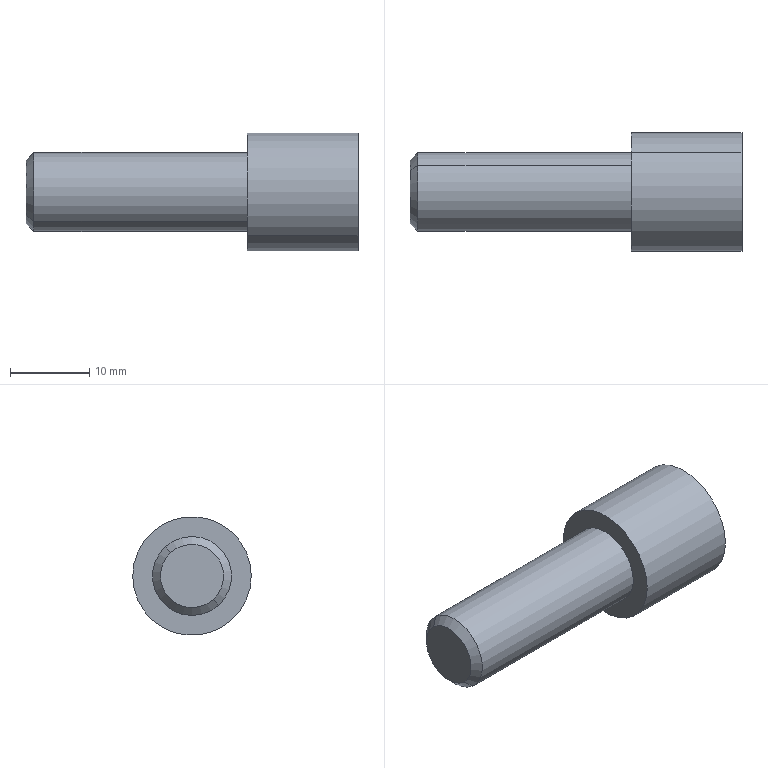Component | SolidWorks | CountersunkScrewM5X20-3 | 1 solid | 16 faces | box 42 x 15 x 15 mm | volume 4378 mm3 | plane 10 | cylinder 4 | cone 2 | commonest cylinder face diameters 10 x2 15 x2
STEP:
#1=COLOUR_RGB('',0.7922,0.8196,0.9333);
#2=FILL_AREA_STYLE_COLOUR('',#1);
#3=FILL_AREA_STYLE('',(#2));
#4=SURFACE_STYLE_FILL_AREA(#3);
#5=SURFACE_SIDE_STYLE('',(#4));
#6=SURFACE_STYLE_USAGE(.BOTH.,#5);
#7=PRESENTATION_STYLE_ASSIGNMENT((#6));
#8=CARTESIAN_POINT('',(-15.906,6.664,0.7501));
#9=VERTEX_POINT('',#8);
#10=CARTESIAN_POINT('',(-15.906,6.875,0.9835));
#11=VERTEX_POINT('',#10);
#12=CARTESIAN_POINT('',(-15.906,6.769,0.8668));
#13=DIRECTION('',(-1.,0.,0.));
#14=DIRECTION('',(0.,-0.6713,-0.7412));
#15=AXIS2_PLACEMENT_3D('',#12,#13,#14);
#16=CIRCLE('',#15,0.1575);
#17=EDGE_CURVE('',#9,#11,#16,.T.);
#18=ORIENTED_EDGE('',*,*,#17,.F.);
#19=CARTESIAN_POINT('',(-15.866,6.637,0.7209));
#20=VERTEX_POINT('',#19);
#21=CARTESIAN_POINT('',(-15.906,6.664,0.7501));
#22=DIRECTION('',(0.7071,-0.4747,-0.5241));
#23=VECTOR('',#22,39.37);
#24=LINE('',#21,#23);
#25=EDGE_CURVE('',#9,#20,#24,.T.);
#26=ORIENTED_EDGE('',*,*,#25,.T.);
#27=CARTESIAN_POINT('',(-15.866,6.902,1.013));
#28=VERTEX_POINT('',#27);
#29=CARTESIAN_POINT('',(-15.866,6.769,0.8668));
#30=DIRECTION('',(1.,-0.,-0.));
#31=DIRECTION('',(0.,-0.6713,-0.7412));
#32=AXIS2_PLACEMENT_3D('',#29,#30,#31);
#33=CIRCLE('',#32,0.1969);
#34=EDGE_CURVE('',#28,#20,#33,.T.);
#35=ORIENTED_EDGE('',*,*,#34,.F.);
#36=CARTESIAN_POINT('',(-15.906,6.875,0.9835));
#37=DIRECTION('',(0.7071,0.4747,0.5241));
#38=VECTOR('',#37,39.37);
#39=LINE('',#36,#38);
#40=EDGE_CURVE('',#11,#28,#39,.T.);
#41=ORIENTED_EDGE('',*,*,#40,.F.);
#42=EDGE_LOOP('',(#18,#26,#35,#41));
#43=FACE_OUTER_BOUND('',#42,.T.);
#44=CARTESIAN_POINT('',(-15.906,6.769,0.8668));
#45=DIRECTION('',(1.,-0.,-0.));
#46=DIRECTION('',(0.,0.6713,0.7412));
#47=AXIS2_PLACEMENT_3D('',#44,#45,#46);
#48=CONICAL_SURFACE('',#47,0.1575,0.7854);
#49=ADVANCED_FACE('',(#43),#48,.T.);
#50=ORIENTED_EDGE('',*,*,#34,.T.);
#51=CARTESIAN_POINT('',(-14.803,6.637,0.7209));
#52=VERTEX_POINT('',#51);
#53=CARTESIAN_POINT('',(-15.906,6.637,0.7209));
#54=DIRECTION('',(1.,-0.,-0.));
#55=VECTOR('',#54,39.37);
#56=LINE('',#53,#55);
#57=EDGE_CURVE('',#20,#52,#56,.T.);
#58=ORIENTED_EDGE('',*,*,#57,.T.);
#59=CARTESIAN_POINT('',(-14.803,6.902,1.013));
#60=VERTEX_POINT('',#59);
#61=CARTESIAN_POINT('',(-14.803,6.769,0.8668));
#62=DIRECTION('',(-1.,0.,0.));
#63=DIRECTION('',(0.,-0.6713,-0.7412));
#64=AXIS2_PLACEMENT_3D('',#61,#62,#63);
#65=CIRCLE('',#64,0.1969);
#66=EDGE_CURVE('',#52,#60,#65,.T.);
#67=ORIENTED_EDGE('',*,*,#66,.T.);
#68=CARTESIAN_POINT('',(-15.906,6.902,1.013));
#69=DIRECTION('',(1.,-0.,-0.));
#70=VECTOR('',#69,39.37);
#71=LINE('',#68,#70);
#72=EDGE_CURVE('',#28,#60,#71,.T.);
#73=ORIENTED_EDGE('',*,*,#72,.F.);
#74=EDGE_LOOP('',(#50,#58,#67,#73));
#75=FACE_OUTER_BOUND('',#74,.T.);
#76=CARTESIAN_POINT('',(-15.906,6.769,0.8668));
#77=DIRECTION('',(1.,-0.,-0.));
#78=DIRECTION('',(0.,0.6713,0.7412));
#79=AXIS2_PLACEMENT_3D('',#76,#77,#78);
#80=CYLINDRICAL_SURFACE('',#79,0.1969);
#81=ADVANCED_FACE('',(#75),#80,.T.);
#82=CARTESIAN_POINT('',(-14.252,6.968,1.086));
#83=VERTEX_POINT('',#82);
#84=CARTESIAN_POINT('',(-14.252,6.571,0.648));
#85=VERTEX_POINT('',#84);
#86=CARTESIAN_POINT('',(-14.252,6.769,0.8668));
#87=DIRECTION('',(1.,-0.,-0.));
#88=DIRECTION('',(0.,0.6713,0.7412));
#89=AXIS2_PLACEMENT_3D('',#86,#87,#88);
#90=CIRCLE('',#89,0.2953);
#91=EDGE_CURVE('',#83,#85,#90,.T.);
#92=ORIENTED_EDGE('',*,*,#91,.F.);
#93=CARTESIAN_POINT('',(-14.803,6.968,1.086));
#94=VERTEX_POINT('',#93);
#95=CARTESIAN_POINT('',(-14.252,6.968,1.086));
#96=DIRECTION('',(-1.,0.,0.));
#97=VECTOR('',#96,39.37);
#98=LINE('',#95,#97);
#99=EDGE_CURVE('',#83,#94,#98,.T.);
#100=ORIENTED_EDGE('',*,*,#99,.T.);
#101=CARTESIAN_POINT('',(-14.803,6.571,0.648));
#102=VERTEX_POINT('',#101);
#103=CARTESIAN_POINT('',(-14.803,6.769,0.8668));
#104=DIRECTION('',(1.,-0.,-0.));
#105=DIRECTION('',(0.,0.6713,0.7412));
#106=AXIS2_PLACEMENT_3D('',#103,#104,#105);
#107=CIRCLE('',#106,0.2953);
#108=EDGE_CURVE('',#94,#102,#107,.T.);
#109=ORIENTED_EDGE('',*,*,#108,.T.);
#110=CARTESIAN_POINT('',(-14.252,6.571,0.648));
#111=DIRECTION('',(-1.,0.,0.));
#112=VECTOR('',#111,39.37);
#113=LINE('',#110,#112);
#114=EDGE_CURVE('',#85,#102,#113,.T.);
#115=ORIENTED_EDGE('',*,*,#114,.F.);
#116=EDGE_LOOP('',(#92,#100,#109,#115));
#117=FACE_OUTER_BOUND('',#116,.T.);
#118=CARTESIAN_POINT('',(-14.252,6.769,0.8668));
#119=DIRECTION('',(-1.,0.,0.));
#120=DIRECTION('',(0.,-0.6713,-0.7412));
#121=AXIS2_PLACEMENT_3D('',#118,#119,#120);
#122=CYLINDRICAL_SURFACE('',#121,0.2953);
#123=ADVANCED_FACE('',(#117),#122,.T.);
#124=ORIENTED_EDGE('',*,*,#99,.F.);
#125=CARTESIAN_POINT('',(-14.252,6.769,0.8668));
#126=DIRECTION('',(1.,-0.,-0.));
#127=DIRECTION('',(0.,0.6713,0.7412));
#128=AXIS2_PLACEMENT_3D('',#125,#126,#127);
#129=CIRCLE('',#128,0.2953);
#130=EDGE_CURVE('',#85,#83,#129,.T.);
#131=ORIENTED_EDGE('',*,*,#130,.F.);
#132=ORIENTED_EDGE('',*,*,#114,.T.);
#133=CARTESIAN_POINT('',(-14.803,6.769,0.8668));
#134=DIRECTION('',(1.,-0.,-0.));
#135=DIRECTION('',(0.,0.6713,0.7412));
#136=AXIS2_PLACEMENT_3D('',#133,#134,#135);
#137=CIRCLE('',#136,0.2953);
#138=EDGE_CURVE('',#102,#94,#137,.T.);
#139=ORIENTED_EDGE('',*,*,#138,.T.);
#140=EDGE_LOOP('',(#124,#131,#132,#139));
#141=FACE_OUTER_BOUND('',#140,.T.);
#142=CARTESIAN_POINT('',(-14.252,6.769,0.8668));
#143=DIRECTION('',(-1.,0.,0.));
#144=DIRECTION('',(0.,-0.6713,-0.7412));
#145=AXIS2_PLACEMENT_3D('',#142,#143,#144);
#146=CYLINDRICAL_SURFACE('',#145,0.2953);
#147=ADVANCED_FACE('',(#141),#146,.T.);
#148=CARTESIAN_POINT('',(-14.252,6.802,1.018));
#149=VERTEX_POINT('',#148);
#150=CARTESIAN_POINT('',(-14.252,6.655,0.9706));
#151=VERTEX_POINT('',#150);
#152=CARTESIAN_POINT('',(-14.252,6.802,1.018));
#153=DIRECTION('',(-0.,-0.952,-0.3062));
#154=VECTOR('',#153,39.37);
#155=LINE('',#152,#154);
#156=EDGE_CURVE('',#149,#151,#155,.T.);
#157=ORIENTED_EDGE('',*,*,#156,.F.);
#158=CARTESIAN_POINT('',(-14.252,6.917,0.9141));
#159=VERTEX_POINT('',#158);
#160=CARTESIAN_POINT('',(-14.252,6.917,0.9141));
#161=DIRECTION('',(0.,-0.7412,0.6713));
#162=VECTOR('',#161,39.37);
#163=LINE('',#160,#162);
#164=EDGE_CURVE('',#159,#149,#163,.T.);
#165=ORIENTED_EDGE('',*,*,#164,.F.);
#166=CARTESIAN_POINT('',(-14.252,6.884,0.763));
#167=VERTEX_POINT('',#166);
#168=CARTESIAN_POINT('',(-14.252,6.884,0.763));
#169=DIRECTION('',(0.,0.2108,0.9775));
#170=VECTOR('',#169,39.37);
#171=LINE('',#168,#170);
#172=EDGE_CURVE('',#167,#159,#171,.T.);
#173=ORIENTED_EDGE('',*,*,#172,.F.);
#174=CARTESIAN_POINT('',(-14.252,6.737,0.7157));
#175=VERTEX_POINT('',#174);
#176=CARTESIAN_POINT('',(-14.252,6.737,0.7157));
#177=DIRECTION('',(0.,0.952,0.3062));
#178=VECTOR('',#177,39.37);
#179=LINE('',#176,#178);
#180=EDGE_CURVE('',#175,#167,#179,.T.);
#181=ORIENTED_EDGE('',*,*,#180,.F.);
#182=CARTESIAN_POINT('',(-14.252,6.622,0.8195));
#183=VERTEX_POINT('',#182);
#184=CARTESIAN_POINT('',(-14.252,6.622,0.8195));
#185=DIRECTION('',(-0.,0.7412,-0.6713));
#186=VECTOR('',#185,39.37);
#187=LINE('',#184,#186);
#188=EDGE_CURVE('',#183,#175,#187,.T.);
#189=ORIENTED_EDGE('',*,*,#188,.F.);
#190=CARTESIAN_POINT('',(-14.252,6.655,0.9706));
#191=DIRECTION('',(-0.,-0.2108,-0.9775));
#192=VECTOR('',#191,39.37);
#193=LINE('',#190,#192);
#194=EDGE_CURVE('',#151,#183,#193,.T.);
#195=ORIENTED_EDGE('',*,*,#194,.F.);
#196=EDGE_LOOP('',(#157,#165,#173,#181,#189,#195));
#197=FACE_BOUND('',#196,.T.);
#198=ORIENTED_EDGE('',*,*,#130,.T.);
#199=ORIENTED_EDGE('',*,*,#91,.T.);
#200=EDGE_LOOP('',(#198,#199));
#201=FACE_OUTER_BOUND('',#200,.T.);
#202=CARTESIAN_POINT('',(-14.252,6.769,0.8668));
#203=DIRECTION('',(1.,-0.,-0.));
#204=DIRECTION('',(0.,0.6713,0.7412));
#205=AXIS2_PLACEMENT_3D('',#202,#203,#204);
#206=PLANE('',#205);
#207=ADVANCED_FACE('',(#197,#201),#206,.T.);
#208=CARTESIAN_POINT('',(-14.803,6.769,0.8668));
#209=DIRECTION('',(-1.,0.,0.));
#210=DIRECTION('',(0.,-0.6713,-0.7412));
#211=AXIS2_PLACEMENT_3D('',#208,#209,#210);
#212=CIRCLE('',#211,0.1969);
#213=EDGE_CURVE('',#60,#52,#212,.T.);
#214=ORIENTED_EDGE('',*,*,#213,.F.);
#215=ORIENTED_EDGE('',*,*,#66,.F.);
#216=EDGE_LOOP('',(#214,#215));
#217=FACE_BOUND('',#216,.T.);
#218=ORIENTED_EDGE('',*,*,#138,.F.);
#219=ORIENTED_EDGE('',*,*,#108,.F.);
#220=EDGE_LOOP('',(#218,#219));
#221=FACE_OUTER_BOUND('',#220,.T.);
#222=CARTESIAN_POINT('',(-14.803,6.769,0.8668));
#223=DIRECTION('',(1.,-0.,-0.));
#224=DIRECTION('',(0.,0.6713,0.7412));
#225=AXIS2_PLACEMENT_3D('',#222,#223,#224);
#226=PLANE('',#225);
#227=ADVANCED_FACE('',(#217,#221),#226,.F.);
#228=ORIENTED_EDGE('',*,*,#57,.F.);
#229=CARTESIAN_POINT('',(-15.866,6.769,0.8668));
#230=DIRECTION('',(1.,-0.,-0.));
#231=DIRECTION('',(0.,-0.6713,-0.7412));
#232=AXIS2_PLACEMENT_3D('',#229,#230,#231);
#233=CIRCLE('',#232,0.1969);
#234=EDGE_CURVE('',#20,#28,#233,.T.);
#235=ORIENTED_EDGE('',*,*,#234,.T.);
#236=ORIENTED_EDGE('',*,*,#72,.T.);
#237=ORIENTED_EDGE('',*,*,#213,.T.);
#238=EDGE_LOOP('',(#228,#235,#236,#237));
#239=FACE_OUTER_BOUND('',#238,.T.);
#240=CARTESIAN_POINT('',(-15.906,6.769,0.8668));
#241=DIRECTION('',(1.,-0.,-0.));
#242=DIRECTION('',(0.,0.6713,0.7412));
#243=AXIS2_PLACEMENT_3D('',#240,#241,#242);
#244=CYLINDRICAL_SURFACE('',#243,0.1969);
#245=ADVANCED_FACE('',(#239),#244,.T.);
#246=CARTESIAN_POINT('',(-15.906,6.769,0.8668));
#247=DIRECTION('',(-1.,0.,0.));
#248=DIRECTION('',(0.,-0.6713,-0.7412));
#249=AXIS2_PLACEMENT_3D('',#246,#247,#248);
#250=CIRCLE('',#249,0.1575);
#251=EDGE_CURVE('',#11,#9,#250,.T.);
#252=ORIENTED_EDGE('',*,*,#251,.T.);
#253=ORIENTED_EDGE('',*,*,#17,.T.);
#254=EDGE_LOOP('',(#252,#253));
#255=FACE_OUTER_BOUND('',#254,.T.);
#256=CARTESIAN_POINT('',(-15.906,6.769,0.8668));
#257=DIRECTION('',(-1.,0.,0.));
#258=DIRECTION('',(-0.,-0.6713,-0.7412));
#259=AXIS2_PLACEMENT_3D('',#256,#257,#258);
#260=PLANE('',#259);
#261=ADVANCED_FACE('',(#255),#260,.T.);
#262=ORIENTED_EDGE('',*,*,#25,.F.);
#263=ORIENTED_EDGE('',*,*,#251,.F.);
#264=ORIENTED_EDGE('',*,*,#40,.T.);
#265=ORIENTED_EDGE('',*,*,#234,.F.);
#266=EDGE_LOOP('',(#262,#263,#264,#265));
#267=FACE_OUTER_BOUND('',#266,.T.);
#268=CARTESIAN_POINT('',(-15.906,6.769,0.8668));
#269=DIRECTION('',(1.,-0.,-0.));
#270=DIRECTION('',(0.,0.6713,0.7412));
#271=AXIS2_PLACEMENT_3D('',#268,#269,#270);
#272=CONICAL_SURFACE('',#271,0.1575,0.7854);
#273=ADVANCED_FACE('',(#267),#272,.T.);
#274=ORIENTED_EDGE('',*,*,#156,.T.);
#275=CARTESIAN_POINT('',(-14.528,6.655,0.9706));
#276=VERTEX_POINT('',#275);
#277=CARTESIAN_POINT('',(-14.528,6.655,0.9706));
#278=DIRECTION('',(1.,-0.,-0.));
#279=VECTOR('',#278,39.37);
#280=LINE('',#277,#279);
#281=EDGE_CURVE('',#276,#151,#280,.T.);
#282=ORIENTED_EDGE('',*,*,#281,.F.);
#283=CARTESIAN_POINT('',(-14.528,6.802,1.018));
#284=VERTEX_POINT('',#283);
#285=CARTESIAN_POINT('',(-14.528,6.802,1.018));
#286=DIRECTION('',(-0.,-0.952,-0.3062));
#287=VECTOR('',#286,39.37);
#288=LINE('',#285,#287);
#289=EDGE_CURVE('',#284,#276,#288,.T.);
#290=ORIENTED_EDGE('',*,*,#289,.F.);
#291=CARTESIAN_POINT('',(-14.528,6.802,1.018));
#292=DIRECTION('',(1.,-0.,-0.));
#293=VECTOR('',#292,39.37);
#294=LINE('',#291,#293);
#295=EDGE_CURVE('',#284,#149,#294,.T.);
#296=ORIENTED_EDGE('',*,*,#295,.T.);
#297=EDGE_LOOP('',(#274,#282,#290,#296));
#298=FACE_OUTER_BOUND('',#297,.T.);
#299=CARTESIAN_POINT('',(-14.528,6.802,1.018));
#300=DIRECTION('',(0.,-0.3062,0.952));
#301=DIRECTION('',(-0.,-0.952,-0.3062));
#302=AXIS2_PLACEMENT_3D('',#299,#300,#301);
#303=PLANE('',#302);
#304=ADVANCED_FACE('',(#298),#303,.F.);
#305=ORIENTED_EDGE('',*,*,#164,.T.);
#306=ORIENTED_EDGE('',*,*,#295,.F.);
#307=CARTESIAN_POINT('',(-14.528,6.917,0.9141));
#308=VERTEX_POINT('',#307);
#309=CARTESIAN_POINT('',(-14.528,6.917,0.9141));
#310=DIRECTION('',(0.,-0.7412,0.6713));
#311=VECTOR('',#310,39.37);
#312=LINE('',#309,#311);
#313=EDGE_CURVE('',#308,#284,#312,.T.);
#314=ORIENTED_EDGE('',*,*,#313,.F.);
#315=CARTESIAN_POINT('',(-14.528,6.917,0.9141));
#316=DIRECTION('',(1.,-0.,-0.));
#317=VECTOR('',#316,39.37);
#318=LINE('',#315,#317);
#319=EDGE_CURVE('',#308,#159,#318,.T.);
#320=ORIENTED_EDGE('',*,*,#319,.T.);
#321=EDGE_LOOP('',(#305,#306,#314,#320));
#322=FACE_OUTER_BOUND('',#321,.T.);
#323=CARTESIAN_POINT('',(-14.528,6.917,0.9141));
#324=DIRECTION('',(0.,0.6713,0.7412));
#325=DIRECTION('',(-1.,0.,0.));
#326=AXIS2_PLACEMENT_3D('',#323,#324,#325);
#327=PLANE('',#326);
#328=ADVANCED_FACE('',(#322),#327,.F.);
#329=ORIENTED_EDGE('',*,*,#172,.T.);
#330=ORIENTED_EDGE('',*,*,#319,.F.);
#331=CARTESIAN_POINT('',(-14.528,6.884,0.763));
#332=VERTEX_POINT('',#331);
#333=CARTESIAN_POINT('',(-14.528,6.884,0.763));
#334=DIRECTION('',(0.,0.2108,0.9775));
#335=VECTOR('',#334,39.37);
#336=LINE('',#333,#335);
#337=EDGE_CURVE('',#332,#308,#336,.T.);
#338=ORIENTED_EDGE('',*,*,#337,.F.);
#339=CARTESIAN_POINT('',(-14.528,6.884,0.763));
#340=DIRECTION('',(1.,-0.,-0.));
#341=VECTOR('',#340,39.37);
#342=LINE('',#339,#341);
#343=EDGE_CURVE('',#332,#167,#342,.T.);
#344=ORIENTED_EDGE('',*,*,#343,.T.);
#345=EDGE_LOOP('',(#329,#330,#338,#344));
#346=FACE_OUTER_BOUND('',#345,.T.);
#347=CARTESIAN_POINT('',(-14.528,6.884,0.763));
#348=DIRECTION('',(0.,0.9775,-0.2108));
#349=DIRECTION('',(0.,0.2108,0.9775));
#350=AXIS2_PLACEMENT_3D('',#347,#348,#349);
#351=PLANE('',#350);
#352=ADVANCED_FACE('',(#346),#351,.F.);
#353=ORIENTED_EDGE('',*,*,#180,.T.);
#354=ORIENTED_EDGE('',*,*,#343,.F.);
#355=CARTESIAN_POINT('',(-14.528,6.737,0.7157));
#356=VERTEX_POINT('',#355);
#357=CARTESIAN_POINT('',(-14.528,6.737,0.7157));
#358=DIRECTION('',(0.,0.952,0.3062));
#359=VECTOR('',#358,39.37);
#360=LINE('',#357,#359);
#361=EDGE_CURVE('',#356,#332,#360,.T.);
#362=ORIENTED_EDGE('',*,*,#361,.F.);
#363=CARTESIAN_POINT('',(-14.528,6.737,0.7157));
#364=DIRECTION('',(1.,-0.,-0.));
#365=VECTOR('',#364,39.37);
#366=LINE('',#363,#365);
#367=EDGE_CURVE('',#356,#175,#366,.T.);
#368=ORIENTED_EDGE('',*,*,#367,.T.);
#369=EDGE_LOOP('',(#353,#354,#362,#368));
#370=FACE_OUTER_BOUND('',#369,.T.);
#371=CARTESIAN_POINT('',(-14.528,6.737,0.7157));
#372=DIRECTION('',(-0.,0.3062,-0.952));
#373=DIRECTION('',(0.,0.952,0.3062));
#374=AXIS2_PLACEMENT_3D('',#371,#372,#373);
#375=PLANE('',#374);
#376=ADVANCED_FACE('',(#370),#375,.F.);
#377=ORIENTED_EDGE('',*,*,#188,.T.);
#378=ORIENTED_EDGE('',*,*,#367,.F.);
#379=CARTESIAN_POINT('',(-14.528,6.622,0.8195));
#380=VERTEX_POINT('',#379);
#381=CARTESIAN_POINT('',(-14.528,6.622,0.8195));
#382=DIRECTION('',(-0.,0.7412,-0.6713));
#383=VECTOR('',#382,39.37);
#384=LINE('',#381,#383);
#385=EDGE_CURVE('',#380,#356,#384,.T.);
#386=ORIENTED_EDGE('',*,*,#385,.F.);
#387=CARTESIAN_POINT('',(-14.528,6.622,0.8195));
#388=DIRECTION('',(1.,-0.,-0.));
#389=VECTOR('',#388,39.37);
#390=LINE('',#387,#389);
#391=EDGE_CURVE('',#380,#183,#390,.T.);
#392=ORIENTED_EDGE('',*,*,#391,.T.);
#393=EDGE_LOOP('',(#377,#378,#386,#392));
#394=FACE_OUTER_BOUND('',#393,.T.);
#395=CARTESIAN_POINT('',(-14.528,6.622,0.8195));
#396=DIRECTION('',(-0.,-0.6713,-0.7412));
#397=DIRECTION('',(1.,-0.,-0.));
#398=AXIS2_PLACEMENT_3D('',#395,#396,#397);
#399=PLANE('',#398);
#400=ADVANCED_FACE('',(#394),#399,.F.);
#401=ORIENTED_EDGE('',*,*,#194,.T.);
#402=ORIENTED_EDGE('',*,*,#391,.F.);
#403=CARTESIAN_POINT('',(-14.528,6.655,0.9706));
#404=DIRECTION('',(-0.,-0.2108,-0.9775));
#405=VECTOR('',#404,39.37);
#406=LINE('',#403,#405);
#407=EDGE_CURVE('',#276,#380,#406,.T.);
#408=ORIENTED_EDGE('',*,*,#407,.F.);
#409=ORIENTED_EDGE('',*,*,#281,.T.);
#410=EDGE_LOOP('',(#401,#402,#408,#409));
#411=FACE_OUTER_BOUND('',#410,.T.);
#412=CARTESIAN_POINT('',(-14.528,6.655,0.9706));
#413=DIRECTION('',(-0.,-0.9775,0.2108));
#414=DIRECTION('',(-0.,-0.2108,-0.9775));
#415=AXIS2_PLACEMENT_3D('',#412,#413,#414);
#416=PLANE('',#415);
#417=ADVANCED_FACE('',(#411),#416,.F.);
#418=ORIENTED_EDGE('',*,*,#289,.T.);
#419=ORIENTED_EDGE('',*,*,#407,.T.);
#420=ORIENTED_EDGE('',*,*,#385,.T.);
#421=ORIENTED_EDGE('',*,*,#361,.T.);
#422=ORIENTED_EDGE('',*,*,#337,.T.);
#423=ORIENTED_EDGE('',*,*,#313,.T.);
#424=EDGE_LOOP('',(#418,#419,#420,#421,#422,#423));
#425=FACE_OUTER_BOUND('',#424,.T.);
#426=CARTESIAN_POINT('',(-14.528,11.691,-4.034));
#427=DIRECTION('',(1.,-0.,-0.));
#428=DIRECTION('',(0.,0.6713,0.7412));
#429=AXIS2_PLACEMENT_3D('',#426,#427,#428);
#430=PLANE('',#429);
#431=ADVANCED_FACE('',(#425),#430,.T.);
#432=CLOSED_SHELL('',(#49,#81,#123,#147,#207,#227,#245,#261,#273,#304,#328,#352,#376,#400,#417,#431));
#433=MANIFOLD_SOLID_BREP('',#432);
#434=STYLED_ITEM('',(#7),#433);
#435=(LENGTH_UNIT()NAMED_UNIT(*)SI_UNIT($,.METRE.));
#436=LENGTH_MEASURE_WITH_UNIT(LENGTH_MEASURE(0.0254),#435);
#437=DIMENSIONAL_EXPONENTS(1.,0.,0.,0.,0.,0.,0.);
#438=(CONVERSION_BASED_UNIT('',#436)LENGTH_UNIT()NAMED_UNIT(#437));
#439=UNCERTAINTY_MEASURE_WITH_UNIT(LENGTH_MEASURE(0.00001),#438,'','');
#440=(NAMED_UNIT(*)PLANE_ANGLE_UNIT()SI_UNIT($,.RADIAN.));
#441=(NAMED_UNIT(*)SI_UNIT($,.STERADIAN.)SOLID_ANGLE_UNIT());
#442=(GEOMETRIC_REPRESENTATION_CONTEXT(3)GLOBAL_UNCERTAINTY_ASSIGNED_CONTEXT((#439))GLOBAL_UNIT_ASSIGNED_CONTEXT((#438,#440,#441))REPRESENTATION_CONTEXT('',''));
#443=MECHANICAL_DESIGN_GEOMETRIC_PRESENTATION_REPRESENTATION('',(#434),#442);
#444=CARTESIAN_POINT('',(0.,0.,0.));
#445=DIRECTION('',(0.,0.,1.));
#446=DIRECTION('',(1.,0.,0.));
#447=AXIS2_PLACEMENT_3D('',#444,#445,#446);
#448=(LENGTH_UNIT()NAMED_UNIT(*)SI_UNIT($,.METRE.));
#449=LENGTH_MEASURE_WITH_UNIT(LENGTH_MEASURE(0.0254),#448);
#450=DIMENSIONAL_EXPONENTS(1.,0.,0.,0.,0.,0.,0.);
#451=(CONVERSION_BASED_UNIT('',#449)LENGTH_UNIT()NAMED_UNIT(#450));
#452=UNCERTAINTY_MEASURE_WITH_UNIT(LENGTH_MEASURE(0.00001),#451,'','');
#453=(NAMED_UNIT(*)PLANE_ANGLE_UNIT()SI_UNIT($,.RADIAN.));
#454=(NAMED_UNIT(*)SI_UNIT($,.STERADIAN.)SOLID_ANGLE_UNIT());
#455=(GEOMETRIC_REPRESENTATION_CONTEXT(3)GLOBAL_UNCERTAINTY_ASSIGNED_CONTEXT((#452))GLOBAL_UNIT_ASSIGNED_CONTEXT((#451,#453,#454))REPRESENTATION_CONTEXT('',''));
#456=ADVANCED_BREP_SHAPE_REPRESENTATION('',(#433,#447),#455);
#457=PRESENTATION_LAYER_ASSIGNMENT('','',(#434));